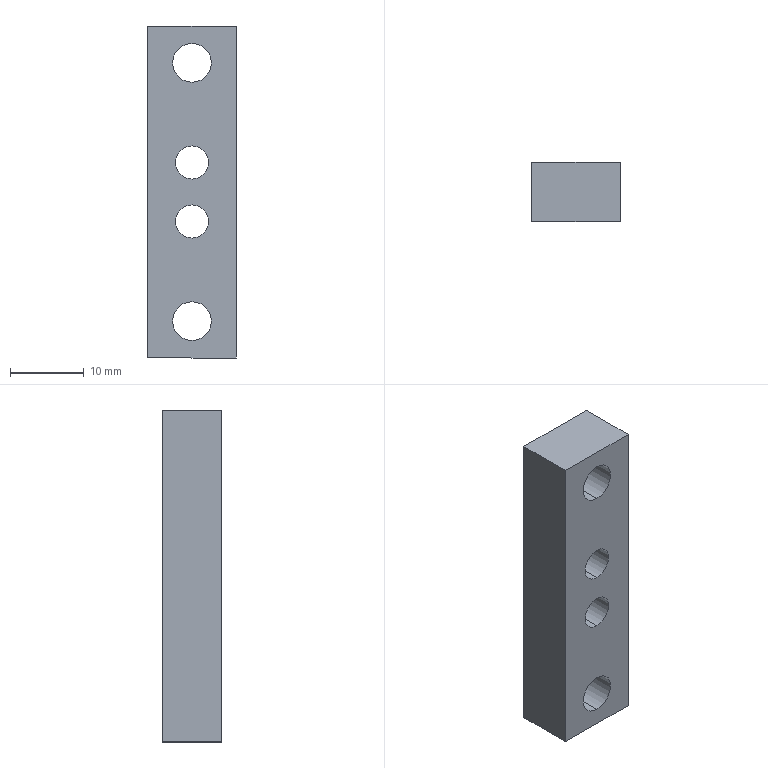Component | SolidWorks | 7.1.02.0001.00.00-0053-1 | 1 solid | 14 faces | box 12 x 8 x 45 mm | volume 3719 mm3 | cylinder 8 | plane 6 | commonest cylinder face diameters 5.25 x4 4.5 x4
build123d program:
from build123d import *

# Parameters (mm, degrees)
SKETCH1_W              = 45
SKETCH1_H              = 12
SKETCH1_R              = 2.25
BOSS_EXTRUDE1_DEPTH    = 8
M6X0_75_TAPPED_HOLE1_D = 5.25


with BuildPart() as part:
    # Sketch1 → Boss-Extrude1 (new body)
    with BuildSketch(Plane.XY):
        Rectangle(SKETCH1_W, SKETCH1_H)
        with Locations((-4, 0)):
            Circle(SKETCH1_R, mode=Mode.SUBTRACT)
        with Locations((4, 0)):
            Circle(SKETCH1_R, mode=Mode.SUBTRACT)
    extrude(amount=BOSS_EXTRUDE1_DEPTH)

    # M6x0.75 Tapped Hole1 (through all)
    with Locations(Plane(origin=(-17.5, 0, 8), x_dir=(1, 0, 0), z_dir=(0, 0, 1))):
        with Locations((0, 0), (35, 0)):
            Hole(M6X0_75_TAPPED_HOLE1_D / 2)


solid = part.part

# Placed as in the assembly
solid = solid.moved(Location((-30.964, 54.316, 0), (90, 0, 90)))
STEP:
#1=CARTESIAN_POINT('',(-1.219,1.823,0.7923));
#2=VERTEX_POINT('',#1);
#3=CARTESIAN_POINT('',(-1.219,1.823,0.5856));
#4=VERTEX_POINT('',#3);
#5=CARTESIAN_POINT('',(-1.219,1.823,0.689));
#6=DIRECTION('',(-0.,1.,-0.));
#7=DIRECTION('',(0.,0.,-1.));
#8=AXIS2_PLACEMENT_3D('',#5,#6,#7);
#9=CIRCLE('',#8,0.1033);
#10=EDGE_CURVE('',#2,#4,#9,.T.);
#11=ORIENTED_EDGE('',*,*,#10,.F.);
#12=CARTESIAN_POINT('',(-1.219,2.138,0.7923));
#13=VERTEX_POINT('',#12);
#14=CARTESIAN_POINT('',(-1.219,2.138,0.7923));
#15=DIRECTION('',(-0.,1.,-0.));
#16=VECTOR('',#15,39.37);
#17=LINE('',#14,#16);
#18=EDGE_CURVE('',#2,#13,#17,.T.);
#19=ORIENTED_EDGE('',*,*,#18,.T.);
#20=CARTESIAN_POINT('',(-1.219,2.138,0.5856));
#21=VERTEX_POINT('',#20);
#22=CARTESIAN_POINT('',(-1.219,2.138,0.689));
#23=DIRECTION('',(-0.,1.,-0.));
#24=DIRECTION('',(0.,0.,-1.));
#25=AXIS2_PLACEMENT_3D('',#22,#23,#24);
#26=CIRCLE('',#25,0.1033);
#27=EDGE_CURVE('',#13,#21,#26,.T.);
#28=ORIENTED_EDGE('',*,*,#27,.T.);
#29=CARTESIAN_POINT('',(-1.219,2.138,0.5856));
#30=DIRECTION('',(-0.,1.,-0.));
#31=VECTOR('',#30,39.37);
#32=LINE('',#29,#31);
#33=EDGE_CURVE('',#4,#21,#32,.T.);
#34=ORIENTED_EDGE('',*,*,#33,.F.);
#35=EDGE_LOOP('',(#11,#19,#28,#34));
#36=FACE_OUTER_BOUND('',#35,.T.);
#37=CARTESIAN_POINT('',(-1.219,2.138,0.689));
#38=DIRECTION('',(-0.,1.,-0.));
#39=DIRECTION('',(0.,0.,-1.));
#40=AXIS2_PLACEMENT_3D('',#37,#38,#39);
#41=CYLINDRICAL_SURFACE('',#40,0.1033);
#42=ADVANCED_FACE('',(#36),#41,.F.);
#43=CARTESIAN_POINT('',(-1.219,1.823,-0.5856));
#44=VERTEX_POINT('',#43);
#45=CARTESIAN_POINT('',(-1.219,1.823,-0.7923));
#46=VERTEX_POINT('',#45);
#47=CARTESIAN_POINT('',(-1.219,1.823,-0.689));
#48=DIRECTION('',(-0.,1.,-0.));
#49=DIRECTION('',(0.,0.,-1.));
#50=AXIS2_PLACEMENT_3D('',#47,#48,#49);
#51=CIRCLE('',#50,0.1033);
#52=EDGE_CURVE('',#44,#46,#51,.T.);
#53=ORIENTED_EDGE('',*,*,#52,.F.);
#54=CARTESIAN_POINT('',(-1.219,2.138,-0.5856));
#55=VERTEX_POINT('',#54);
#56=CARTESIAN_POINT('',(-1.219,2.138,-0.5856));
#57=DIRECTION('',(-0.,1.,-0.));
#58=VECTOR('',#57,39.37);
#59=LINE('',#56,#58);
#60=EDGE_CURVE('',#44,#55,#59,.T.);
#61=ORIENTED_EDGE('',*,*,#60,.T.);
#62=CARTESIAN_POINT('',(-1.219,2.138,-0.7923));
#63=VERTEX_POINT('',#62);
#64=CARTESIAN_POINT('',(-1.219,2.138,-0.689));
#65=DIRECTION('',(-0.,1.,-0.));
#66=DIRECTION('',(0.,0.,-1.));
#67=AXIS2_PLACEMENT_3D('',#64,#65,#66);
#68=CIRCLE('',#67,0.1033);
#69=EDGE_CURVE('',#55,#63,#68,.T.);
#70=ORIENTED_EDGE('',*,*,#69,.T.);
#71=CARTESIAN_POINT('',(-1.219,2.138,-0.7923));
#72=DIRECTION('',(-0.,1.,-0.));
#73=VECTOR('',#72,39.37);
#74=LINE('',#71,#73);
#75=EDGE_CURVE('',#46,#63,#74,.T.);
#76=ORIENTED_EDGE('',*,*,#75,.F.);
#77=EDGE_LOOP('',(#53,#61,#70,#76));
#78=FACE_OUTER_BOUND('',#77,.T.);
#79=CARTESIAN_POINT('',(-1.219,2.138,-0.689));
#80=DIRECTION('',(-0.,1.,-0.));
#81=DIRECTION('',(0.,0.,-1.));
#82=AXIS2_PLACEMENT_3D('',#79,#80,#81);
#83=CYLINDRICAL_SURFACE('',#82,0.1033);
#84=ADVANCED_FACE('',(#78),#83,.F.);
#85=CARTESIAN_POINT('',(-1.219,2.138,-0.0689));
#86=VERTEX_POINT('',#85);
#87=CARTESIAN_POINT('',(-1.219,2.138,-0.2461));
#88=VERTEX_POINT('',#87);
#89=CARTESIAN_POINT('',(-1.219,2.138,-0.1575));
#90=DIRECTION('',(-0.,1.,-0.));
#91=DIRECTION('',(0.,0.,-1.));
#92=AXIS2_PLACEMENT_3D('',#89,#90,#91);
#93=CIRCLE('',#92,0.08858);
#94=EDGE_CURVE('',#86,#88,#93,.T.);
#95=ORIENTED_EDGE('',*,*,#94,.T.);
#96=CARTESIAN_POINT('',(-1.219,1.823,-0.2461));
#97=VERTEX_POINT('',#96);
#98=CARTESIAN_POINT('',(-1.219,2.138,-0.2461));
#99=DIRECTION('',(0.,-1.,0.));
#100=VECTOR('',#99,39.37);
#101=LINE('',#98,#100);
#102=EDGE_CURVE('',#88,#97,#101,.T.);
#103=ORIENTED_EDGE('',*,*,#102,.T.);
#104=CARTESIAN_POINT('',(-1.219,1.823,-0.0689));
#105=VERTEX_POINT('',#104);
#106=CARTESIAN_POINT('',(-1.219,1.823,-0.1575));
#107=DIRECTION('',(-0.,1.,-0.));
#108=DIRECTION('',(0.,0.,-1.));
#109=AXIS2_PLACEMENT_3D('',#106,#107,#108);
#110=CIRCLE('',#109,0.08858);
#111=EDGE_CURVE('',#105,#97,#110,.T.);
#112=ORIENTED_EDGE('',*,*,#111,.F.);
#113=CARTESIAN_POINT('',(-1.219,2.138,-0.0689));
#114=DIRECTION('',(0.,-1.,0.));
#115=VECTOR('',#114,39.37);
#116=LINE('',#113,#115);
#117=EDGE_CURVE('',#86,#105,#116,.T.);
#118=ORIENTED_EDGE('',*,*,#117,.F.);
#119=EDGE_LOOP('',(#95,#103,#112,#118));
#120=FACE_OUTER_BOUND('',#119,.T.);
#121=CARTESIAN_POINT('',(-1.219,2.138,-0.1575));
#122=DIRECTION('',(0.,-1.,0.));
#123=DIRECTION('',(0.,0.,1.));
#124=AXIS2_PLACEMENT_3D('',#121,#122,#123);
#125=CYLINDRICAL_SURFACE('',#124,0.08858);
#126=ADVANCED_FACE('',(#120),#125,.F.);
#127=CARTESIAN_POINT('',(-1.219,2.138,0.2461));
#128=VERTEX_POINT('',#127);
#129=CARTESIAN_POINT('',(-1.219,2.138,0.0689));
#130=VERTEX_POINT('',#129);
#131=CARTESIAN_POINT('',(-1.219,2.138,0.1575));
#132=DIRECTION('',(-0.,1.,-0.));
#133=DIRECTION('',(0.,0.,-1.));
#134=AXIS2_PLACEMENT_3D('',#131,#132,#133);
#135=CIRCLE('',#134,0.08858);
#136=EDGE_CURVE('',#128,#130,#135,.T.);
#137=ORIENTED_EDGE('',*,*,#136,.T.);
#138=CARTESIAN_POINT('',(-1.219,1.823,0.0689));
#139=VERTEX_POINT('',#138);
#140=CARTESIAN_POINT('',(-1.219,2.138,0.0689));
#141=DIRECTION('',(0.,-1.,0.));
#142=VECTOR('',#141,39.37);
#143=LINE('',#140,#142);
#144=EDGE_CURVE('',#130,#139,#143,.T.);
#145=ORIENTED_EDGE('',*,*,#144,.T.);
#146=CARTESIAN_POINT('',(-1.219,1.823,0.2461));
#147=VERTEX_POINT('',#146);
#148=CARTESIAN_POINT('',(-1.219,1.823,0.1575));
#149=DIRECTION('',(-0.,1.,-0.));
#150=DIRECTION('',(0.,0.,-1.));
#151=AXIS2_PLACEMENT_3D('',#148,#149,#150);
#152=CIRCLE('',#151,0.08858);
#153=EDGE_CURVE('',#147,#139,#152,.T.);
#154=ORIENTED_EDGE('',*,*,#153,.F.);
#155=CARTESIAN_POINT('',(-1.219,2.138,0.2461));
#156=DIRECTION('',(0.,-1.,0.));
#157=VECTOR('',#156,39.37);
#158=LINE('',#155,#157);
#159=EDGE_CURVE('',#128,#147,#158,.T.);
#160=ORIENTED_EDGE('',*,*,#159,.F.);
#161=EDGE_LOOP('',(#137,#145,#154,#160));
#162=FACE_OUTER_BOUND('',#161,.T.);
#163=CARTESIAN_POINT('',(-1.219,2.138,0.1575));
#164=DIRECTION('',(0.,-1.,0.));
#165=DIRECTION('',(0.,0.,1.));
#166=AXIS2_PLACEMENT_3D('',#163,#164,#165);
#167=CYLINDRICAL_SURFACE('',#166,0.08858);
#168=ADVANCED_FACE('',(#162),#167,.F.);
#169=CARTESIAN_POINT('',(-1.219,2.138,0.689));
#170=DIRECTION('',(-0.,1.,-0.));
#171=DIRECTION('',(0.,0.,-1.));
#172=AXIS2_PLACEMENT_3D('',#169,#170,#171);
#173=CIRCLE('',#172,0.1033);
#174=EDGE_CURVE('',#21,#13,#173,.T.);
#175=ORIENTED_EDGE('',*,*,#174,.F.);
#176=ORIENTED_EDGE('',*,*,#27,.F.);
#177=EDGE_LOOP('',(#175,#176));
#178=FACE_BOUND('',#177,.T.);
#179=CARTESIAN_POINT('',(-1.219,2.138,-0.689));
#180=DIRECTION('',(-0.,1.,-0.));
#181=DIRECTION('',(0.,0.,-1.));
#182=AXIS2_PLACEMENT_3D('',#179,#180,#181);
#183=CIRCLE('',#182,0.1033);
#184=EDGE_CURVE('',#63,#55,#183,.T.);
#185=ORIENTED_EDGE('',*,*,#184,.F.);
#186=ORIENTED_EDGE('',*,*,#69,.F.);
#187=EDGE_LOOP('',(#185,#186));
#188=FACE_BOUND('',#187,.T.);
#189=ORIENTED_EDGE('',*,*,#136,.F.);
#190=CARTESIAN_POINT('',(-1.219,2.138,0.1575));
#191=DIRECTION('',(-0.,1.,-0.));
#192=DIRECTION('',(0.,0.,-1.));
#193=AXIS2_PLACEMENT_3D('',#190,#191,#192);
#194=CIRCLE('',#193,0.08858);
#195=EDGE_CURVE('',#130,#128,#194,.T.);
#196=ORIENTED_EDGE('',*,*,#195,.F.);
#197=EDGE_LOOP('',(#189,#196));
#198=FACE_BOUND('',#197,.T.);
#199=CARTESIAN_POINT('',(-1.455,2.138,0.8858));
#200=VERTEX_POINT('',#199);
#201=CARTESIAN_POINT('',(-0.9828,2.138,0.8858));
#202=VERTEX_POINT('',#201);
#203=CARTESIAN_POINT('',(-1.455,2.138,0.8858));
#204=DIRECTION('',(1.,-0.,-0.));
#205=VECTOR('',#204,39.37);
#206=LINE('',#203,#205);
#207=EDGE_CURVE('',#200,#202,#206,.T.);
#208=ORIENTED_EDGE('',*,*,#207,.T.);
#209=CARTESIAN_POINT('',(-0.9828,2.138,-0.8858));
#210=VERTEX_POINT('',#209);
#211=CARTESIAN_POINT('',(-0.9828,2.138,0.8858));
#212=DIRECTION('',(-0.,0.,-1.));
#213=VECTOR('',#212,39.37);
#214=LINE('',#211,#213);
#215=EDGE_CURVE('',#202,#210,#214,.T.);
#216=ORIENTED_EDGE('',*,*,#215,.T.);
#217=CARTESIAN_POINT('',(-1.455,2.138,-0.8858));
#218=VERTEX_POINT('',#217);
#219=CARTESIAN_POINT('',(-1.455,2.138,-0.8858));
#220=DIRECTION('',(-1.,0.,0.));
#221=VECTOR('',#220,39.37);
#222=LINE('',#219,#221);
#223=EDGE_CURVE('',#210,#218,#222,.T.);
#224=ORIENTED_EDGE('',*,*,#223,.T.);
#225=CARTESIAN_POINT('',(-1.455,2.138,0.8858));
#226=DIRECTION('',(0.,-0.,1.));
#227=VECTOR('',#226,39.37);
#228=LINE('',#225,#227);
#229=EDGE_CURVE('',#218,#200,#228,.T.);
#230=ORIENTED_EDGE('',*,*,#229,.T.);
#231=EDGE_LOOP('',(#208,#216,#224,#230));
#232=FACE_OUTER_BOUND('',#231,.T.);
#233=ORIENTED_EDGE('',*,*,#94,.F.);
#234=CARTESIAN_POINT('',(-1.219,2.138,-0.1575));
#235=DIRECTION('',(-0.,1.,-0.));
#236=DIRECTION('',(0.,0.,-1.));
#237=AXIS2_PLACEMENT_3D('',#234,#235,#236);
#238=CIRCLE('',#237,0.08858);
#239=EDGE_CURVE('',#88,#86,#238,.T.);
#240=ORIENTED_EDGE('',*,*,#239,.F.);
#241=EDGE_LOOP('',(#233,#240));
#242=FACE_BOUND('',#241,.T.);
#243=CARTESIAN_POINT('',(-1.219,2.138,-0.));
#244=DIRECTION('',(-0.,1.,0.));
#245=DIRECTION('',(-0.,0.,-1.));
#246=AXIS2_PLACEMENT_3D('',#243,#244,#245);
#247=PLANE('',#246);
#248=ADVANCED_FACE('',(#178,#188,#198,#232,#242),#247,.T.);
#249=CARTESIAN_POINT('',(-1.219,1.823,0.689));
#250=DIRECTION('',(-0.,1.,-0.));
#251=DIRECTION('',(0.,0.,-1.));
#252=AXIS2_PLACEMENT_3D('',#249,#250,#251);
#253=CIRCLE('',#252,0.1033);
#254=EDGE_CURVE('',#4,#2,#253,.T.);
#255=ORIENTED_EDGE('',*,*,#254,.T.);
#256=ORIENTED_EDGE('',*,*,#10,.T.);
#257=EDGE_LOOP('',(#255,#256));
#258=FACE_BOUND('',#257,.T.);
#259=CARTESIAN_POINT('',(-1.219,1.823,-0.689));
#260=DIRECTION('',(-0.,1.,-0.));
#261=DIRECTION('',(0.,0.,-1.));
#262=AXIS2_PLACEMENT_3D('',#259,#260,#261);
#263=CIRCLE('',#262,0.1033);
#264=EDGE_CURVE('',#46,#44,#263,.T.);
#265=ORIENTED_EDGE('',*,*,#264,.T.);
#266=ORIENTED_EDGE('',*,*,#52,.T.);
#267=EDGE_LOOP('',(#265,#266));
#268=FACE_BOUND('',#267,.T.);
#269=ORIENTED_EDGE('',*,*,#153,.T.);
#270=CARTESIAN_POINT('',(-1.219,1.823,0.1575));
#271=DIRECTION('',(-0.,1.,-0.));
#272=DIRECTION('',(0.,0.,-1.));
#273=AXIS2_PLACEMENT_3D('',#270,#271,#272);
#274=CIRCLE('',#273,0.08858);
#275=EDGE_CURVE('',#139,#147,#274,.T.);
#276=ORIENTED_EDGE('',*,*,#275,.T.);
#277=EDGE_LOOP('',(#269,#276));
#278=FACE_BOUND('',#277,.T.);
#279=CARTESIAN_POINT('',(-1.455,1.823,0.8858));
#280=VERTEX_POINT('',#279);
#281=CARTESIAN_POINT('',(-0.9828,1.823,0.8858));
#282=VERTEX_POINT('',#281);
#283=CARTESIAN_POINT('',(-1.455,1.823,0.8858));
#284=DIRECTION('',(1.,-0.,-0.));
#285=VECTOR('',#284,39.37);
#286=LINE('',#283,#285);
#287=EDGE_CURVE('',#280,#282,#286,.T.);
#288=ORIENTED_EDGE('',*,*,#287,.F.);
#289=CARTESIAN_POINT('',(-1.455,1.823,-0.8858));
#290=VERTEX_POINT('',#289);
#291=CARTESIAN_POINT('',(-1.455,1.823,0.8858));
#292=DIRECTION('',(0.,-0.,1.));
#293=VECTOR('',#292,39.37);
#294=LINE('',#291,#293);
#295=EDGE_CURVE('',#290,#280,#294,.T.);
#296=ORIENTED_EDGE('',*,*,#295,.F.);
#297=CARTESIAN_POINT('',(-0.9828,1.823,-0.8858));
#298=VERTEX_POINT('',#297);
#299=CARTESIAN_POINT('',(-1.455,1.823,-0.8858));
#300=DIRECTION('',(-1.,0.,0.));
#301=VECTOR('',#300,39.37);
#302=LINE('',#299,#301);
#303=EDGE_CURVE('',#298,#290,#302,.T.);
#304=ORIENTED_EDGE('',*,*,#303,.F.);
#305=CARTESIAN_POINT('',(-0.9828,1.823,0.8858));
#306=DIRECTION('',(-0.,0.,-1.));
#307=VECTOR('',#306,39.37);
#308=LINE('',#305,#307);
#309=EDGE_CURVE('',#282,#298,#308,.T.);
#310=ORIENTED_EDGE('',*,*,#309,.F.);
#311=EDGE_LOOP('',(#288,#296,#304,#310));
#312=FACE_OUTER_BOUND('',#311,.T.);
#313=ORIENTED_EDGE('',*,*,#111,.T.);
#314=CARTESIAN_POINT('',(-1.219,1.823,-0.1575));
#315=DIRECTION('',(-0.,1.,-0.));
#316=DIRECTION('',(0.,0.,-1.));
#317=AXIS2_PLACEMENT_3D('',#314,#315,#316);
#318=CIRCLE('',#317,0.08858);
#319=EDGE_CURVE('',#97,#105,#318,.T.);
#320=ORIENTED_EDGE('',*,*,#319,.T.);
#321=EDGE_LOOP('',(#313,#320));
#322=FACE_BOUND('',#321,.T.);
#323=CARTESIAN_POINT('',(-1.219,1.823,-0.));
#324=DIRECTION('',(-0.,1.,0.));
#325=DIRECTION('',(-0.,0.,-1.));
#326=AXIS2_PLACEMENT_3D('',#323,#324,#325);
#327=PLANE('',#326);
#328=ADVANCED_FACE('',(#258,#268,#278,#312,#322),#327,.F.);
#329=ORIENTED_EDGE('',*,*,#287,.T.);
#330=CARTESIAN_POINT('',(-0.9828,2.138,0.8858));
#331=DIRECTION('',(0.,-1.,0.));
#332=VECTOR('',#331,39.37);
#333=LINE('',#330,#332);
#334=EDGE_CURVE('',#202,#282,#333,.T.);
#335=ORIENTED_EDGE('',*,*,#334,.F.);
#336=ORIENTED_EDGE('',*,*,#207,.F.);
#337=CARTESIAN_POINT('',(-1.455,2.138,0.8858));
#338=DIRECTION('',(0.,-1.,0.));
#339=VECTOR('',#338,39.37);
#340=LINE('',#337,#339);
#341=EDGE_CURVE('',#200,#280,#340,.T.);
#342=ORIENTED_EDGE('',*,*,#341,.T.);
#343=EDGE_LOOP('',(#329,#335,#336,#342));
#344=FACE_OUTER_BOUND('',#343,.T.);
#345=CARTESIAN_POINT('',(-1.455,2.138,0.8858));
#346=DIRECTION('',(-0.,-0.,-1.));
#347=DIRECTION('',(0.,-1.,0.));
#348=AXIS2_PLACEMENT_3D('',#345,#346,#347);
#349=PLANE('',#348);
#350=ADVANCED_FACE('',(#344),#349,.F.);
#351=ORIENTED_EDGE('',*,*,#309,.T.);
#352=CARTESIAN_POINT('',(-0.9828,2.138,-0.8858));
#353=DIRECTION('',(0.,-1.,0.));
#354=VECTOR('',#353,39.37);
#355=LINE('',#352,#354);
#356=EDGE_CURVE('',#210,#298,#355,.T.);
#357=ORIENTED_EDGE('',*,*,#356,.F.);
#358=ORIENTED_EDGE('',*,*,#215,.F.);
#359=ORIENTED_EDGE('',*,*,#334,.T.);
#360=EDGE_LOOP('',(#351,#357,#358,#359));
#361=FACE_OUTER_BOUND('',#360,.T.);
#362=CARTESIAN_POINT('',(-0.9828,2.138,0.8858));
#363=DIRECTION('',(-1.,-0.,0.));
#364=DIRECTION('',(-0.,1.,-0.));
#365=AXIS2_PLACEMENT_3D('',#362,#363,#364);
#366=PLANE('',#365);
#367=ADVANCED_FACE('',(#361),#366,.F.);
#368=ORIENTED_EDGE('',*,*,#303,.T.);
#369=CARTESIAN_POINT('',(-1.455,2.138,-0.8858));
#370=DIRECTION('',(0.,-1.,0.));
#371=VECTOR('',#370,39.37);
#372=LINE('',#369,#371);
#373=EDGE_CURVE('',#218,#290,#372,.T.);
#374=ORIENTED_EDGE('',*,*,#373,.F.);
#375=ORIENTED_EDGE('',*,*,#223,.F.);
#376=ORIENTED_EDGE('',*,*,#356,.T.);
#377=EDGE_LOOP('',(#368,#374,#375,#376));
#378=FACE_OUTER_BOUND('',#377,.T.);
#379=CARTESIAN_POINT('',(-1.455,2.138,-0.8858));
#380=DIRECTION('',(0.,0.,1.));
#381=DIRECTION('',(-0.,1.,-0.));
#382=AXIS2_PLACEMENT_3D('',#379,#380,#381);
#383=PLANE('',#382);
#384=ADVANCED_FACE('',(#378),#383,.F.);
#385=ORIENTED_EDGE('',*,*,#295,.T.);
#386=ORIENTED_EDGE('',*,*,#341,.F.);
#387=ORIENTED_EDGE('',*,*,#229,.F.);
#388=ORIENTED_EDGE('',*,*,#373,.T.);
#389=EDGE_LOOP('',(#385,#386,#387,#388));
#390=FACE_OUTER_BOUND('',#389,.T.);
#391=CARTESIAN_POINT('',(-1.455,2.138,0.8858));
#392=DIRECTION('',(1.,0.,-0.));
#393=DIRECTION('',(0.,-1.,0.));
#394=AXIS2_PLACEMENT_3D('',#391,#392,#393);
#395=PLANE('',#394);
#396=ADVANCED_FACE('',(#390),#395,.F.);
#397=ORIENTED_EDGE('',*,*,#144,.F.);
#398=ORIENTED_EDGE('',*,*,#195,.T.);
#399=ORIENTED_EDGE('',*,*,#159,.T.);
#400=ORIENTED_EDGE('',*,*,#275,.F.);
#401=EDGE_LOOP('',(#397,#398,#399,#400));
#402=FACE_OUTER_BOUND('',#401,.T.);
#403=CARTESIAN_POINT('',(-1.219,2.138,0.1575));
#404=DIRECTION('',(0.,-1.,0.));
#405=DIRECTION('',(0.,0.,1.));
#406=AXIS2_PLACEMENT_3D('',#403,#404,#405);
#407=CYLINDRICAL_SURFACE('',#406,0.08858);
#408=ADVANCED_FACE('',(#402),#407,.F.);
#409=ORIENTED_EDGE('',*,*,#102,.F.);
#410=ORIENTED_EDGE('',*,*,#239,.T.);
#411=ORIENTED_EDGE('',*,*,#117,.T.);
#412=ORIENTED_EDGE('',*,*,#319,.F.);
#413=EDGE_LOOP('',(#409,#410,#411,#412));
#414=FACE_OUTER_BOUND('',#413,.T.);
#415=CARTESIAN_POINT('',(-1.219,2.138,-0.1575));
#416=DIRECTION('',(0.,-1.,0.));
#417=DIRECTION('',(0.,0.,1.));
#418=AXIS2_PLACEMENT_3D('',#415,#416,#417);
#419=CYLINDRICAL_SURFACE('',#418,0.08858);
#420=ADVANCED_FACE('',(#414),#419,.F.);
#421=ORIENTED_EDGE('',*,*,#60,.F.);
#422=ORIENTED_EDGE('',*,*,#264,.F.);
#423=ORIENTED_EDGE('',*,*,#75,.T.);
#424=ORIENTED_EDGE('',*,*,#184,.T.);
#425=EDGE_LOOP('',(#421,#422,#423,#424));
#426=FACE_OUTER_BOUND('',#425,.T.);
#427=CARTESIAN_POINT('',(-1.219,2.138,-0.689));
#428=DIRECTION('',(-0.,1.,-0.));
#429=DIRECTION('',(0.,0.,-1.));
#430=AXIS2_PLACEMENT_3D('',#427,#428,#429);
#431=CYLINDRICAL_SURFACE('',#430,0.1033);
#432=ADVANCED_FACE('',(#426),#431,.F.);
#433=ORIENTED_EDGE('',*,*,#18,.F.);
#434=ORIENTED_EDGE('',*,*,#254,.F.);
#435=ORIENTED_EDGE('',*,*,#33,.T.);
#436=ORIENTED_EDGE('',*,*,#174,.T.);
#437=EDGE_LOOP('',(#433,#434,#435,#436));
#438=FACE_OUTER_BOUND('',#437,.T.);
#439=CARTESIAN_POINT('',(-1.219,2.138,0.689));
#440=DIRECTION('',(-0.,1.,-0.));
#441=DIRECTION('',(0.,0.,-1.));
#442=AXIS2_PLACEMENT_3D('',#439,#440,#441);
#443=CYLINDRICAL_SURFACE('',#442,0.1033);
#444=ADVANCED_FACE('',(#438),#443,.F.);
#445=CLOSED_SHELL('',(#42,#84,#126,#168,#248,#328,#350,#367,#384,#396,#408,#420,#432,#444));
#446=MANIFOLD_SOLID_BREP('',#445);
#447=CARTESIAN_POINT('',(0.,0.,0.));
#448=DIRECTION('',(0.,0.,1.));
#449=DIRECTION('',(1.,0.,0.));
#450=AXIS2_PLACEMENT_3D('',#447,#448,#449);
#451=(LENGTH_UNIT()NAMED_UNIT(*)SI_UNIT($,.METRE.));
#452=LENGTH_MEASURE_WITH_UNIT(LENGTH_MEASURE(0.0254),#451);
#453=DIMENSIONAL_EXPONENTS(1.,0.,0.,0.,0.,0.,0.);
#454=(CONVERSION_BASED_UNIT('',#452)LENGTH_UNIT()NAMED_UNIT(#453));
#455=UNCERTAINTY_MEASURE_WITH_UNIT(LENGTH_MEASURE(0.00001),#454,'','');
#456=(NAMED_UNIT(*)PLANE_ANGLE_UNIT()SI_UNIT($,.RADIAN.));
#457=(NAMED_UNIT(*)SI_UNIT($,.STERADIAN.)SOLID_ANGLE_UNIT());
#458=(GEOMETRIC_REPRESENTATION_CONTEXT(3)GLOBAL_UNCERTAINTY_ASSIGNED_CONTEXT((#455))GLOBAL_UNIT_ASSIGNED_CONTEXT((#454,#456,#457))REPRESENTATION_CONTEXT('',''));
#459=ADVANCED_BREP_SHAPE_REPRESENTATION('',(#446,#450),#458);
#460=COLOUR_RGB('',0.7922,0.8196,0.9333);
#461=FILL_AREA_STYLE_COLOUR('',#460);
#462=FILL_AREA_STYLE('',(#461));
#463=SURFACE_STYLE_FILL_AREA(#462);
#464=SURFACE_SIDE_STYLE('',(#463));
#465=SURFACE_STYLE_USAGE(.BOTH.,#464);
#466=PRESENTATION_STYLE_ASSIGNMENT((#465));
#467=STYLED_ITEM('',(#466),#446);
#468=PRESENTATION_LAYER_ASSIGNMENT('','',(#467));
#469=(LENGTH_UNIT()NAMED_UNIT(*)SI_UNIT($,.METRE.));
#470=LENGTH_MEASURE_WITH_UNIT(LENGTH_MEASURE(0.0254),#469);
#471=DIMENSIONAL_EXPONENTS(1.,0.,0.,0.,0.,0.,0.);
#472=(CONVERSION_BASED_UNIT('',#470)LENGTH_UNIT()NAMED_UNIT(#471));
#473=UNCERTAINTY_MEASURE_WITH_UNIT(LENGTH_MEASURE(0.00001),#472,'','');
#474=(NAMED_UNIT(*)PLANE_ANGLE_UNIT()SI_UNIT($,.RADIAN.));
#475=(NAMED_UNIT(*)SI_UNIT($,.STERADIAN.)SOLID_ANGLE_UNIT());
#476=(GEOMETRIC_REPRESENTATION_CONTEXT(3)GLOBAL_UNCERTAINTY_ASSIGNED_CONTEXT((#473))GLOBAL_UNIT_ASSIGNED_CONTEXT((#472,#474,#475))REPRESENTATION_CONTEXT('',''));
#477=MECHANICAL_DESIGN_GEOMETRIC_PRESENTATION_REPRESENTATION('',(#467),#476);